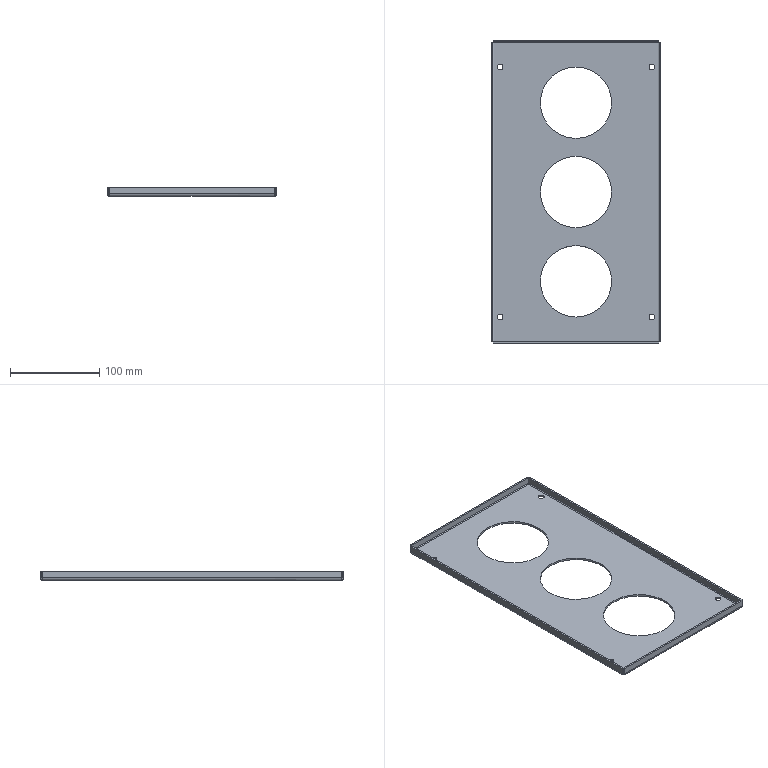Component | SolidWorks | BottomCoverPlate(No.13)-1 | 1 solid | 52 faces | volume 113628 mm3 | cylinder 22 | plane 22 | spline 8 | commonest cylinder face diameters 6.5 x8 80 x6 6 x4 2 x4 | material Plain Carbon Steel